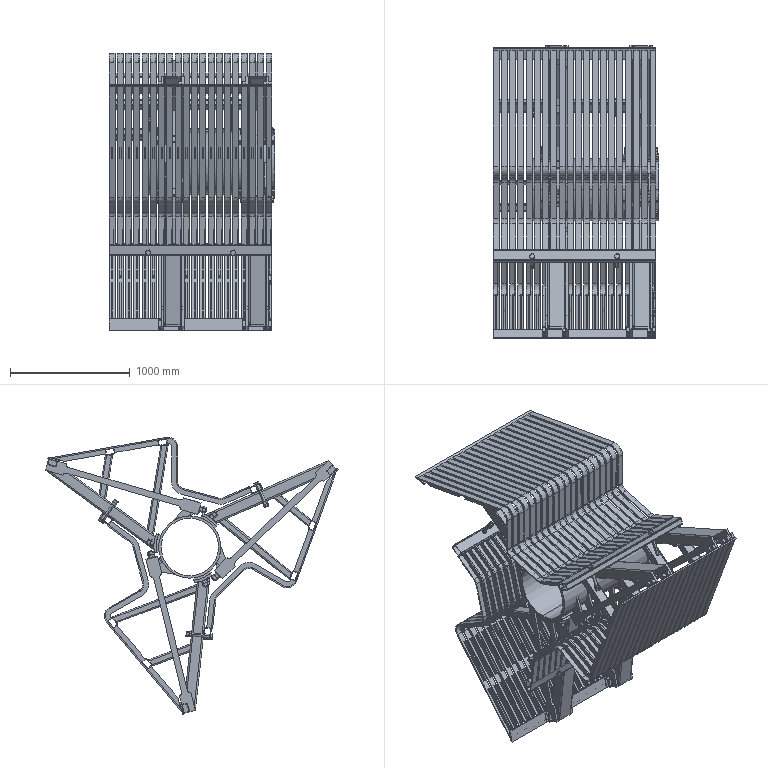Assembly | SolidWorks | mm | 422 component files | 424 solids | 5850 faces | box 1384.6 x 2449.46 x 2319.88 mm | volume 219649083 mm3 | plane 3492 | cylinder 1638 | cone 696 | spline 24 | commonest cylinder face diameters 140 x420 120 x180 30 x132 220 x120 60 x108 19.05 x84 9.525 x84 160 x60
Bill of materials:
Bocna spona oslonca izbacivaca | 12 |  | Thin flat dog-bone strip: a long narrow middle section with a wider rectangular tab at each end, joined by curved transitions.
Cev-osnovna | 1 |  | Straight thin-walled round tube, open at both ends, with plain square-cut ends.
33.7 x 3.2x60 | 6 |  | Short, plain cylindrical tube (hollow sleeve) with a concentric through-bore and flat, square-cut ends.
33.7 x 3.2x100 | 6 |  | Plain cylindrical tube with a concentric through-bore and flat ends. It is longer and more slender than unnamed part.
Donja kontaktna ploca | 6 |  | Curved plate of constant thickness, bent along an arc across its width, with two countersunk through-holes near the ends.
Vijak donje oslone ploce | 12 |  | Plain solid round rod or pin with flat ends.
Donja ploca spone | 6 |  | Curved plate of constant thickness, bent along an arc across its width, with two plain cylindrical through-holes near the ends.
ISO - 4034 - M24 - N | 12 |  | Hexagonal nut-like body with a central smooth round through-bore. It is relatively tall: the axial height is close to the across-flats width. The corners are chamfered on both end faces.
ISO - 4034 - M30 - N | 36 |  | Hexagonal nut-like body with a central smooth round through-bore. It is thinner than unnamed part: the height is noticeably less than the across-flats width. The corners are chamfered on both end faces.
ISO 7412 - M30 x 120 --- 56-WN | 6 |  | Hex-head bolt-like part with a short, plain cylindrical shank. The hex head has chamfered corners, and the shank ends in a flat face with a chamfer.
ISO 7412 - M24 x 200 --- 48-WN | 6 |  | Slender hex-head bolt-like part with a long, plain cylindrical shank. The head is small relative to the shank length, with chamfered hex corners, and the shank end is chamfered.
Oslona ploca izbacivaca | 6 |  | Thick rectangular block-like plate with one round through-hole and a bevel along one edge.
Poprecna spona 1360mm | 3 | Plain Carbon Steel | Long straight rectangular hollow tube with rounded corners and open ends, with two small round holes in one face spaced along its length.
Rebro oslonca izbacivaca | 12 |  | Flat plate of constant thickness with a four-sided outline: three straight edges and one concave curved edge, tapering to a point at one end.
Rebro sipke-1 | 60 |  | Slender straight rectangular bar with one square-cut end and one end cut at an angle.
Rebro sipke-2 | 60 |  | Slender straight rectangular bar with square-cut ends and no other features.
Rebro sipke-3 | 60 |  | Slender member of constant cross-section bent in one plane: several straight segments joined by radiused bends, ending in a short hook-like curl.
rectangular tube_iso | 21 |  | Short closed rectangular band or ring with rounded corners and uniform wall thickness, open through its axis.
SAV1 | 2 |  | Straight prism with a roughly triangular cross-section: two flat sides meet a third side that curves inward. The curved side is built from narrow flat facets.
SAV2 | 2 |  | Solid bar with a rectangular cross-section. Both ends are cut at an angle rather than square.
Sipka resetke | 60 |  | Thin flat strip of constant width, bent into a zig-zag profile with several rounded bends. It has a short end tab, a middle offset section and a long straight leg.
Spona | 6 | Plain Carbon Steel | Thin-walled rectangular tube with rounded corners. One small round hole goes through a broad face. The ends are shaped: one end is cut slightly at an angle with a curved edge, and the other end tapers to a point with a step or notch.
Stap-1 | 6 | Plain Carbon Steel | Straight thin-walled rectangular tube with rounded corners. One end is square and the other is cut at an angle.
Stap-2 | 6 | Plain Carbon Steel | Straight thin-walled rectangular tube with rounded corners. One end is square and the other is cut at an angle. It is shorter for its cross-section size than unnamed part.
Vezni lim 1 | 3 |  | Long, thin, flat rectangular strip with square-cut ends.
Zatezna ploca | 6 |  | Rectangular plate or block with one round through-hole in the center. The top perimeter edges are cut back by wide bevels, and a short vertical edge band sits below them.
Mates:
1. coincident | Oslona ploca izbacivaca-1 face at (0, 225.6, -130.25) dir (1, 0, 0) | assembly plane at (0, 0, 0) dir (1, 0, 0)
2. perpendicular | Oslona ploca izbacivaca-1 edge at (0, 351.871, -161.16) dir (0, -0.9713, 0.2378) | assembly sketch segment at (0, 0, -1390) dir (0, 0.2378, 0.9713)
3. coincident | Zatezna ploca-1 face at (-151, 366.138, -102.881) dir (0, 0.2378, 0.9713) | Bocna spona oslonca izbacivaca-1 face at (21, 366.138, -102.881) dir (0, 0.2378, 0.9713)
4. coincident | Zatezna ploca-1 face at (1, 232.733, -101.11) dir (1, 0, 0) | Bocna spona oslonca izbacivaca-1 face at (1, 98.648, -1216.64) dir (-1, 0, 0)
5. coincident | Zatezna ploca-1 face at (-151, 261.872, -108.243) dir (0, -0.9713, 0.2378) | Bocna spona oslonca izbacivaca-1 face at (21, 233.34, -224.802) dir (0, -0.9713, 0.2378)
6. coincident | Bocna spona oslonca izbacivaca-1 face at (21, 86.758, -1244.184) dir (0, 0.9713, -0.2378) | rectangular tube_iso-2 face at (21, 53.357, -1380.63) dir (0, 0.9713, -0.2378)
7. coincident | Bocna spona oslonca izbacivaca-1 face at (21, 98.648, -1216.64) dir (1, 0, 0) | rectangular tube_iso-2 face at (21, 44.106, -1378.365) dir (-1, 0, 0)
8. coincident | Bocna spona oslonca izbacivaca-1 face at (21, 51.093, -1389.882) dir (0, -0.2378, -0.9713) | rectangular tube_iso-2 face at (21, 41.841, -1387.617) dir (0, -0.2378, -0.9713)
9. coincident | Bocna spona oslonca izbacivaca-1 face at (21, 86.758, -1244.184) dir (0, 0.9713, -0.2378) | rectangular tube_iso-6 face at (-24.4, 53.357, -1380.63) dir (0, 0.9713, -0.2378)
10. coincident | Bocna spona oslonca izbacivaca-1 face at (21, 51.093, -1389.882) dir (0, -0.2378, -0.9713) | rectangular tube_iso-6 face at (-24.4, 41.841, -1387.617) dir (0, -0.2378, -0.9713)
11. coincident | Bocna spona oslonca izbacivaca-1 face at (1, 98.648, -1216.64) dir (-1, 0, 0) | rectangular tube_iso-6 face at (1, 26.855, -1315.305) dir (1, 0, 0)
12. coincident | Cev-osnovna-1 plane at (7660, 0, 0) dir (0, 1, 0) | assembly plane at (0, 0, 0) dir (0, 1, 0)
13. coincident | Cev-osnovna-1 plane at (7660, 0, 0) dir (0, 0, -1) | assembly plane at (0, 0, 0) dir (0, 0, 1)
14. tangent | Cev-osnovna-1 face at (-1000, 0, 0) dir (1, 0, 0) r 260.5 | Donja oslona ploca-2/Donja kontaktna ploca-1 face at (-230, 0, 0) dir (1, 0, 0) r 260.5
15. distance | Donja oslona ploca-2 plane at (-80, -111.051, -257.581) dir (1, 0, 0) | assembly plane at (0, 0, 0) dir (1, 0, 0)
16. coincident | Donja oslona ploca-2/Donja kontaktna ploca-1 face at (70, 0, 0) dir (1, 0, 0) | Donja ploca spone-1 face at (70, 0, 0) dir (1, 0, 0)
17. tangent | Donja oslona ploca-2/Donja kontaktna ploca-1 face at (-230, 0, 0) dir (1, 0, 0) r 280.5 | Donja ploca spone-1 face at (-230, 0, 0) dir (1, 0, 0) r 280.5
18. concentric | Donja oslona ploca-2/Vijak donje oslone ploce-1 face at (33, -142.723, -331.044) dir (0, 0.3959, 0.9183) r 15 | Donja ploca spone-1 face at (33, -118.969, -275.947) dir (0, 0.3959, 0.9183) r 16
19. coincident | Bocna spona oslonca izbacivaca-1 face at (1, 98.648, -1216.64) dir (-1, 0, 0) | Spona-1 face at (1, 0, 0) dir (1, 0, 0)
20. distance | Zatezna ploca-3 face at (-151, -272.166, -265.644) dir (0, 0.7223, -0.6916) | Donja ploca spone-1 edge at (-230, -187.377, -234.926) dir (1, 0, 0)
21. tangent | Donja ploca spone-1 face at (-230, 0, 0) dir (1, 0, 0) r 300.5 | Spona-1 face at (-149, 0, 0) dir (1, 0, 0) r 300.5
22. coincident | Donja ploca spone-1 face at (-230, 0, 0) dir (1, 0, 0) r 300.5 | Spona-1 edge at (-136.4, -167.547, -249.456) dir (1, 0, 0)
23. distance | Spona-1 edge at (-136.4, -62.108, -294.012) dir (1, 0, 0) | Stap-1-1 edge at (-114, -59.945, -313.894) dir (1, 0, 0)
24. distance | Spona-1 face at (1, 0, 0) dir (1, 0, 0) | Stap-1-1 face at (-24, 39.364, -6.624) dir (1, 0, 0)
25. distance | Stap-2-1 face at (-24, 776.667, -2903.89) dir (1, 0, 0) | Spona-1 face at (1, 0, 0) dir (1, 0, 0)
26. coincident | Spona-1 face at (-149, -62.108, -294.012) dir (0, 0.9941, 0.1082) | Stap-2-1 edge at (-34, -6.043, -809.246) dir (-1, 0, 0)
27. concentric | Oslona ploca izbacivaca-1 face at (-75, 303.305, -149.272) dir (0, 0.2378, 0.9713) r 16 | hex structural bolt gradec short_iso-2 face at (-75, 298.859, -167.435) dir (0, -0.2378, -0.9713) r 15
28. coincident | Oslona ploca izbacivaca-1 face at (0, 225.6, -130.25) dir (0, -0.2378, -0.9713) | hex structural bolt gradec short_iso-2 face at (-81.864, 330.541, -155.939) dir (0, 0.2378, 0.9713)
29. concentric | Oslona ploca izbacivaca-9 face at (-785, 303.305, -149.272) dir (0, 0.2378, 0.9713) r 16 | hex structural bolt gradec short_iso-3 face at (-785, 298.859, -167.435) dir (0, -0.2378, -0.9713) r 15
30. coincident | Oslona ploca izbacivaca-9 face at (-710, 225.6, -130.25) dir (0, -0.2378, -0.9713) | hex structural bolt gradec short_iso-3 face at (-791.864, 330.541, -155.939) dir (0, 0.2378, 0.9713)
31. concentric | circular tube_iso-7 face at (-988.6, 699.202, 272.049) dir (0, 0.5907, -0.8069) r 13.65 | hex structural bolt gradec short_iso-4 face at (-988.6, 743.508, 211.535) dir (0, 0.5907, -0.8069) r 12
32. concentric | circular tube_iso-1 face at (-278.6, 699.202, 272.049) dir (0, 0.5907, -0.8069) r 13.65 | hex structural bolt gradec short_iso-5 face at (-278.6, 743.508, 211.535) dir (0, 0.5907, -0.8069) r 12
33. coincident | hex nut gradec_iso-6 face at (-121, 323.849, -65.349) dir (0, 0.2378, 0.9713) | hex nut gradec_iso-7 face at (-121, 323.849, -65.349) dir (0, -0.2378, -0.9713)
34. coincident | Spona-2 face at (-149, 285.676, 93.218) dir (0, -0.5907, 0.8069) | hex nut gradec_iso-8 face at (-83.382, 655.285, 363.833) dir (0, 0.5907, -0.8069)
35. coincident | hex nut gradec_iso-9 face at (-988.6, 611.041, 357.278) dir (0, -0.5907, 0.8069) | hex nut gradec_iso-10 face at (-988.6, 644.581, 381.835) dir (0, 0.5907, -0.8069)
36. coincident | hex nut gradec_iso-8 face at (-83.382, 642.112, 381.826) dir (0, -0.5907, 0.8069) | hex nut gradec_iso-11 face at (-74, 643.918, 383.148) dir (0, 0.5907, -0.8069)
37. coincident | hex nut gradec_iso-16 face at (-13, -129.421, -300.19) dir (0, -0.3959, -0.9183) | hex nut gradec_iso-17 face at (-13, -129.421, -300.19) dir (0, 0.3959, 0.9183)
38. coincident | rectangular tube_iso-2 face at (46.4, 44.106, -1378.365) dir (1, 0, 0) | Vezni lim 1-1 face at (46.4, -13.794, -1219.569) dir (1, 0, 0)
39. coincident | rectangular tube_iso-2 face at (21, 53.357, -1380.63) dir (0, 0.9713, -0.2378) | Vezni lim 1-1 face at (-1313.6, 48.715, -1399.595) dir (0, -0.9713, 0.2378)
40. distance | Vezni lim 1-1 face at (-1313.6, 48.715, -1399.595) dir (0, -0.2378, -0.9713) | rectangular tube_iso-2 face at (21, 41.841, -1387.617) dir (0, -0.2378, -0.9713)
41. coincident | Sipka resetke-1 face at (-3.6, 45.788, -1387.311) dir (0, -0.7661, 0.6427) | rectangular tube_iso-60 face at (46.4, 682.365, -628.489) dir (0, 0.7661, -0.6427)
42. coincident | Sipka resetke-1 face at (46.4, 634.859, -576.203) dir (1, 0, 0) | rectangular tube_iso-60 face at (46.4, 675.068, -622.368) dir (1, 0, 0)
43. coincident | Vezni lim 1-1 face at (46.4, -13.794, -1219.569) dir (1, 0, 0) | Sipka resetke-1 face at (46.4, 634.859, -576.203) dir (1, 0, 0)
44. coincident | Sipka resetke-1 face at (-3.6, 45.788, -1387.311) dir (0, -0.7661, 0.6427) | rectangular tube_iso-63 face at (46.4, 395.593, -970.331) dir (0, 0.7661, -0.6427)
45. coincident | Sipka resetke-1 face at (46.4, 634.859, -576.203) dir (1, 0, 0) | rectangular tube_iso-63 face at (46.4, 388.296, -964.21) dir (1, 0, 0)
46. distance | rectangular tube_iso-63 face at (46.4, 394.417, -956.912) dir (0, 0.6427, 0.7661) | Stap-2-1 edge at (-34, 347.371, -943.551) dir (-1, 0, 0)
47. coincident | Sipka resetke-1 edge at (-3.6, 688.487, -621.192) dir (1, 0, 0) | rectangular tube_iso-60 face at (46.4, 681.19, -615.07) dir (0, 0.6427, 0.7661)
48. distance | rectangular tube_iso-63 face at (46.4, 394.417, -956.912) dir (0, 0.6427, 0.7661) | rectangular tube_iso-60 face at (46.4, 607.892, -653.043) dir (0, -0.6427, -0.7661)
49. coincident | Sipka resetke-1 face at (-3.6, 45.788, -1387.311) dir (0, -0.7661, 0.6427) | Rebro sipke-2-1 face at (16.4, 639.513, -679.57) dir (0, 0.7661, -0.6427)
50. coincident | rectangular tube_iso-60 face at (46.4, 607.892, -653.043) dir (0, -0.6427, -0.7661) | Rebro sipke-2-1 face at (16.4, 608.868, -653.862) dir (0, 0.6427, 0.7661)
51. distance | Rebro sipke-2-1 face at (26.4, -52.445, -1277.205) dir (1, 0, 0) | Sipka resetke-1 face at (46.4, 634.859, -576.203) dir (1, 0, 0)
52. coincident | Spona-1 face at (-149, -62.108, -294.012) dir (0, 0.9941, 0.1082) | Stap-1-1 face at (-124, -52.659, -380.849) dir (0, -0.9941, -0.1082)
53. coincident | rectangular tube_iso-63 face at (46.4, 321.119, -994.885) dir (0, -0.6427, -0.7661) | Rebro sipke-1-43 face at (26.4, 322.096, -995.704) dir (0, 0.6427, 0.7661)
54. coincident | Sipka resetke-1 face at (-3.6, 45.788, -1387.311) dir (0, -0.7661, 0.6427) | Rebro sipke-1-43 face at (26.4, 352.741, -1021.412) dir (0, 0.7661, -0.6427)
55. distance | Rebro sipke-1-43 face at (26.4, 322.096, -995.704) dir (1, 0, 0) | Sipka resetke-1 face at (46.4, 634.859, -576.203) dir (1, 0, 0)
56. coincident | Sipka resetke-1 face at (-3.6, 492.714, 46.503) dir (0, -0.5907, 0.8069) | Rebro sipke-3-43 face at (36.4, 678.167, 182.285) dir (0, 0.5907, -0.8069)
57. coincident | Vezni lim 1-1 face at (-1313.6, 48.715, -1399.595) dir (0, -0.9713, 0.2378) | rectangular tube_iso-54 face at (-906.4, 53.357, -1380.63) dir (0, 0.9713, -0.2378)
58. coincident | Bocna spona oslonca izbacivaca-20 face at (-881, 98.648, -1216.64) dir (-1, 0, 0) | rectangular tube_iso-54 face at (-881, 44.106, -1378.365) dir (1, 0, 0)
59. coincident | rectangular tube_iso-2 face at (21, 41.841, -1387.617) dir (0, -0.2378, -0.9713) | rectangular tube_iso-54 face at (-906.4, 41.841, -1387.617) dir (0, -0.2378, -0.9713)
60. coincident | Bocna spona oslonca izbacivaca-2 face at (-171, 98.648, -1216.64) dir (-1, 0, 0) | rectangular tube_iso-57 face at (-171, 44.106, -1378.365) dir (1, 0, 0)
61. coincident | Vezni lim 1-1 face at (-1313.6, 48.715, -1399.595) dir (0, -0.9713, 0.2378) | rectangular tube_iso-57 face at (-196.4, 53.357, -1380.63) dir (0, 0.9713, -0.2378)
62. coincident | rectangular tube_iso-2 face at (21, 41.841, -1387.617) dir (0, -0.2378, -0.9713) | rectangular tube_iso-57 face at (-196.4, 41.841, -1387.617) dir (0, -0.2378, -0.9713)
63. coincident | Spona-2 face at (-149, 299.809, -20.372) dir (0, 0.5907, -0.8069) | circular tube_iso-1 face at (-278.6, 699.202, 272.049) dir (0, -0.5907, 0.8069)
64. coincident | Spona-8 face at (-859, 299.809, -20.372) dir (0, 0.5907, -0.8069) | circular tube_iso-7 face at (-988.6, 699.202, 272.049) dir (0, -0.5907, 0.8069)
65. concentric | Spona-2 face at (-74, 640.321, 352.876) dir (0, 0.5907, -0.8069) r 17 | circular tube_iso-10 face at (-74, 640.321, 352.876) dir (0, 0.5907, -0.8069) r 16.85
66. concentric | Spona-8 face at (-784, 640.321, 352.876) dir (0, 0.5907, -0.8069) r 17 | circular tube_iso-13 face at (-784, 640.321, 352.876) dir (0, 0.5907, -0.8069) r 16.85
67. coincident | Spona-2 face at (-149, 299.809, -20.372) dir (0, 0.5907, -0.8069) | circular tube_iso-10 face at (-74, 699.396, 272.191) dir (0, 0.5907, -0.8069)
68. coincident | Spona-8 face at (-859, 299.809, -20.372) dir (0, 0.5907, -0.8069) | circular tube_iso-13 face at (-784, 699.396, 272.191) dir (0, 0.5907, -0.8069)
69. coincident | Spona-2 face at (-149, 299.809, -20.372) dir (0, 0.5907, -0.8069) | Poprecna spona 1360mm-48 face at (-1313.6, 715.339, 283.864) dir (0, -0.5907, 0.8069)
70. coincident | hex structural bolt gradec short_iso-4 face at (-981.571, 716.409, 210.284) dir (0, -0.5907, 0.8069) | Poprecna spona 1360mm-48 face at (-1313.6, 750.784, 235.452) dir (0, 0.5907, -0.8069)
71. coincident | hex structural bolt gradec short_iso-5 face at (-264.616, 750.058, 234.92) dir (0, -0.5907, 0.8069) | Poprecna spona 1360mm-48 face at (-1313.6, 750.784, 235.452) dir (0, 0.5907, -0.8069)
72. coincident | rectangular tube_iso-2 face at (46.4, 44.106, -1378.365) dir (1, 0, 0) | Poprecna spona 1360mm-48 face at (46.4, 656.698, 228.535) dir (1, 0, 0)
73. coincident | Sipka resetke-1 face at (-3.6, 492.714, 46.503) dir (0, -0.5907, 0.8069) | Poprecna spona 1360mm-48 face at (-1313.6, 750.784, 235.452) dir (0, 0.5907, -0.8069)
74. concentric | circular tube_iso-1 face at (-278.6, 699.202, 272.049) dir (0, 0.5907, -0.8069) r 16.85 | Poprecna spona 1360mm-48 face at (-278.6, 734.647, 223.638) dir (0, -0.5907, 0.8069) r 17
75. concentric | circular tube_iso-7 face at (-988.6, 699.202, 272.049) dir (0, 0.5907, -0.8069) r 16.85 | Poprecna spona 1360mm-48 face at (-988.6, 734.647, 223.638) dir (0, -0.5907, 0.8069) r 17
76. distance | Spona-2 edge at (-136.4, 299.809, -20.372) dir (1, 0, 0) | Poprecna spona 1360mm-48 face at (-1313.6, 648.63, 222.628) dir (0, -0.8069, -0.5907)
77. coincident | Oslona ploca izbacivaca-1 edge at (0, 225.6, -130.25) dir (-1, 0, 0) | assembly sketch point at (0, 225.6, -130.25) dir (1, 0, 0)
78. concentric | hex structural bolt gradec short_iso-3 face at (-785, 298.859, -167.435) dir (0, -0.2378, -0.9713) r 15 | hex nut gradec_iso-4 edge at (-785, 323.849, -65.349) dir (0, -0.2378, -0.9713) r 15
79. concentric | hex structural bolt gradec short_iso-3 face at (-785, 298.859, -167.435) dir (0, -0.2378, -0.9713) r 15 | hex nut gradec_iso-5 edge at (-785, 330.126, -39.707) dir (0, -0.2378, -0.9713) r 15
80. concentric | hex structural bolt gradec short_iso-2 face at (-75, 298.859, -167.435) dir (0, -0.2378, -0.9713) r 15 | hex nut gradec_iso-6 edge at (-75, 323.849, -65.349) dir (0, -0.2378, -0.9713) r 15
81. concentric | hex nut gradec_iso-6 edge at (-75, 323.849, -65.349) dir (0, -0.2378, -0.9713) r 15 | hex nut gradec_iso-7 edge at (-75, 323.849, -65.349) dir (0, 0.2378, 0.9713) r 15
82. concentric | Spona-2 face at (-74, 640.321, 352.876) dir (0, 0.5907, -0.8069) r 17 | hex nut gradec_iso-8 edge at (-74, 640.321, 352.876) dir (0, -0.5907, 0.8069) r 12
83. concentric | hex structural bolt gradec short_iso-4 face at (-988.6, 743.508, 211.535) dir (0, 0.5907, -0.8069) r 12 | hex nut gradec_iso-9 edge at (-988.6, 627.811, 369.556) dir (0, 0.5907, -0.8069) r 12
84. concentric | hex nut gradec_iso-9 face at (-988.6, 627.811, 369.556) dir (0, -0.5907, 0.8069) r 1047.198 | hex nut gradec_iso-10 edge at (-988.6, 627.811, 369.556) dir (0, -0.5907, 0.8069) r 12
85. concentric | hex nut gradec_iso-8 edge at (-74, 627.147, 370.869) dir (0, -0.5907, 0.8069) r 12 | hex nut gradec_iso-11 edge at (-74, 627.147, 370.869) dir (0, -0.5907, 0.8069) r 12
86. concentric | Donja oslona ploca-2/Vijak donje oslone ploce-1 face at (33, -142.723, -331.044) dir (0, 0.3959, 0.9183) r 15 | hex nut gradec_iso-16 edge at (33, -129.421, -300.19) dir (0, 0.3959, 0.9183) r 15
87. concentric | hex nut gradec_iso-16 edge at (33, -129.421, -300.19) dir (0, 0.3959, 0.9183) r 15 | hex nut gradec_iso-17 edge at (33, -129.421, -300.19) dir (0, -0.3959, -0.9183) r 15
88. concentric | Donja oslona ploca-2/Vijak donje oslone ploce-2 face at (-193, -142.723, -331.044) dir (0, 0.3959, 0.9183) r 15 | hex nut gradec_iso-18 edge at (-193, -129.421, -300.19) dir (0, 0.3959, 0.9183) r 15
89. concentric | Donja oslona ploca-2/Vijak donje oslone ploce-2 face at (-193, -142.723, -331.044) dir (0, 0.3959, 0.9183) r 15 | hex nut gradec_iso-19 edge at (-193, -139.873, -324.433) dir (0, 0.3959, 0.9183) r 15
90. concentric | Donja oslona ploca-10/Vijak donje oslone ploce-1 face at (-677, -142.723, -331.044) dir (0, 0.3959, 0.9183) r 15 | hex nut gradec_iso-20 edge at (-677, -129.421, -300.19) dir (0, 0.3959, 0.9183) r 15
91. concentric | Donja oslona ploca-10/Vijak donje oslone ploce-1 face at (-677, -142.723, -331.044) dir (0, 0.3959, 0.9183) r 15 | hex nut gradec_iso-21 edge at (-677, -139.873, -324.433) dir (0, 0.3959, 0.9183) r 15
92. concentric | Donja oslona ploca-10/Vijak donje oslone ploce-2 face at (-903, -142.723, -331.044) dir (0, 0.3959, 0.9183) r 15 | hex nut gradec_iso-22 edge at (-903, -129.421, -300.19) dir (0, 0.3959, 0.9183) r 15
93. concentric | Donja oslona ploca-10/Vijak donje oslone ploce-2 face at (-903, -142.723, -331.044) dir (0, 0.3959, 0.9183) r 15 | hex nut gradec_iso-23 edge at (-903, -139.873, -324.433) dir (0, 0.3959, 0.9183) r 15
94. coincident | Sipka resetke-1 face at (46.4, 634.859, -576.203) dir (1, 0, 0) | Rebro sipke-3-43 face at (46.4, 634.859, -576.203) dir (1, 0, 0)
95. coincident | Rebro sipke-3-43 face at (36.4, 654.537, 214.559) dir (0, 0.8069, 0.5907) | Poprecna spona 1360mm-48 face at (-1313.6, 648.63, 222.628) dir (0, -0.8069, -0.5907)
96. concentric | Donja kontaktna ploca-1 face at (-113, 0, 30.523) dir (0, 0, -1) r 15 | Vijak donje oslone ploce-2 face at (-113, 0, -80) dir (0, 0, 1) r 15
97. concentric | Donja kontaktna ploca-1 face at (113, 0, 30.523) dir (0, 0, -1) r 15 | Vijak donje oslone ploce-1 face at (113, 0, -80) dir (0, 0, 1) r 15
98. tangent | Donja kontaktna ploca-1 face at (-150, 0, 280.5) dir (1, 0, 0) r 260.5 | Vijak donje oslone ploce-2 face at (-113, 0, 20) dir (0, 0, 1)
99. tangent | Donja kontaktna ploca-1 face at (-150, 0, 280.5) dir (1, 0, 0) r 260.5 | Vijak donje oslone ploce-1 face at (113, 0, 20) dir (0, 0, 1)